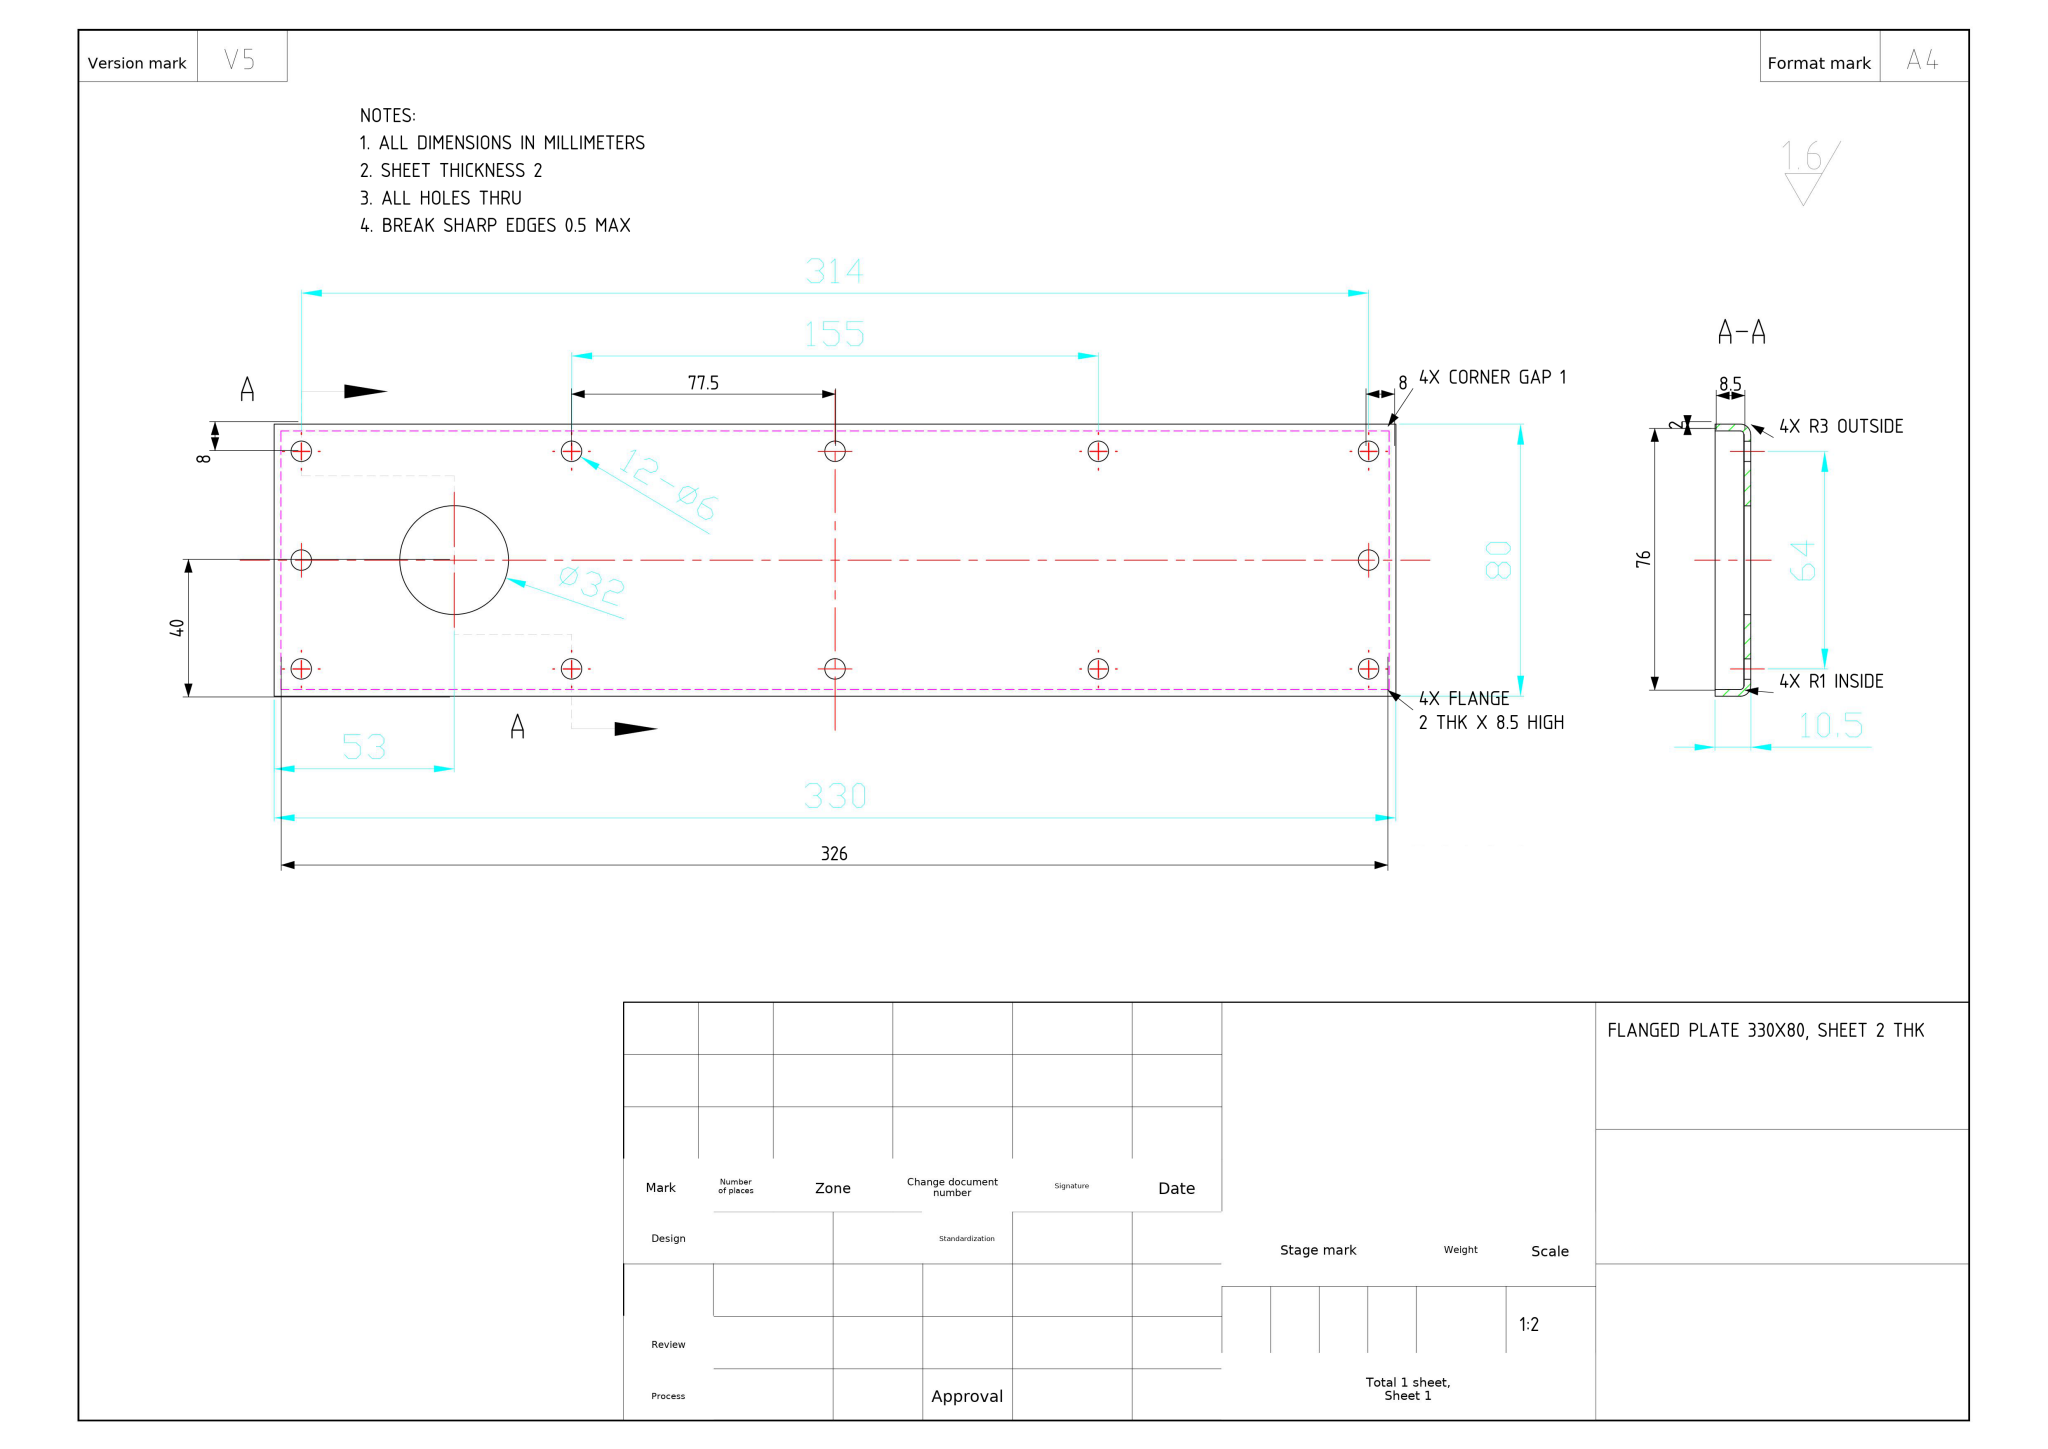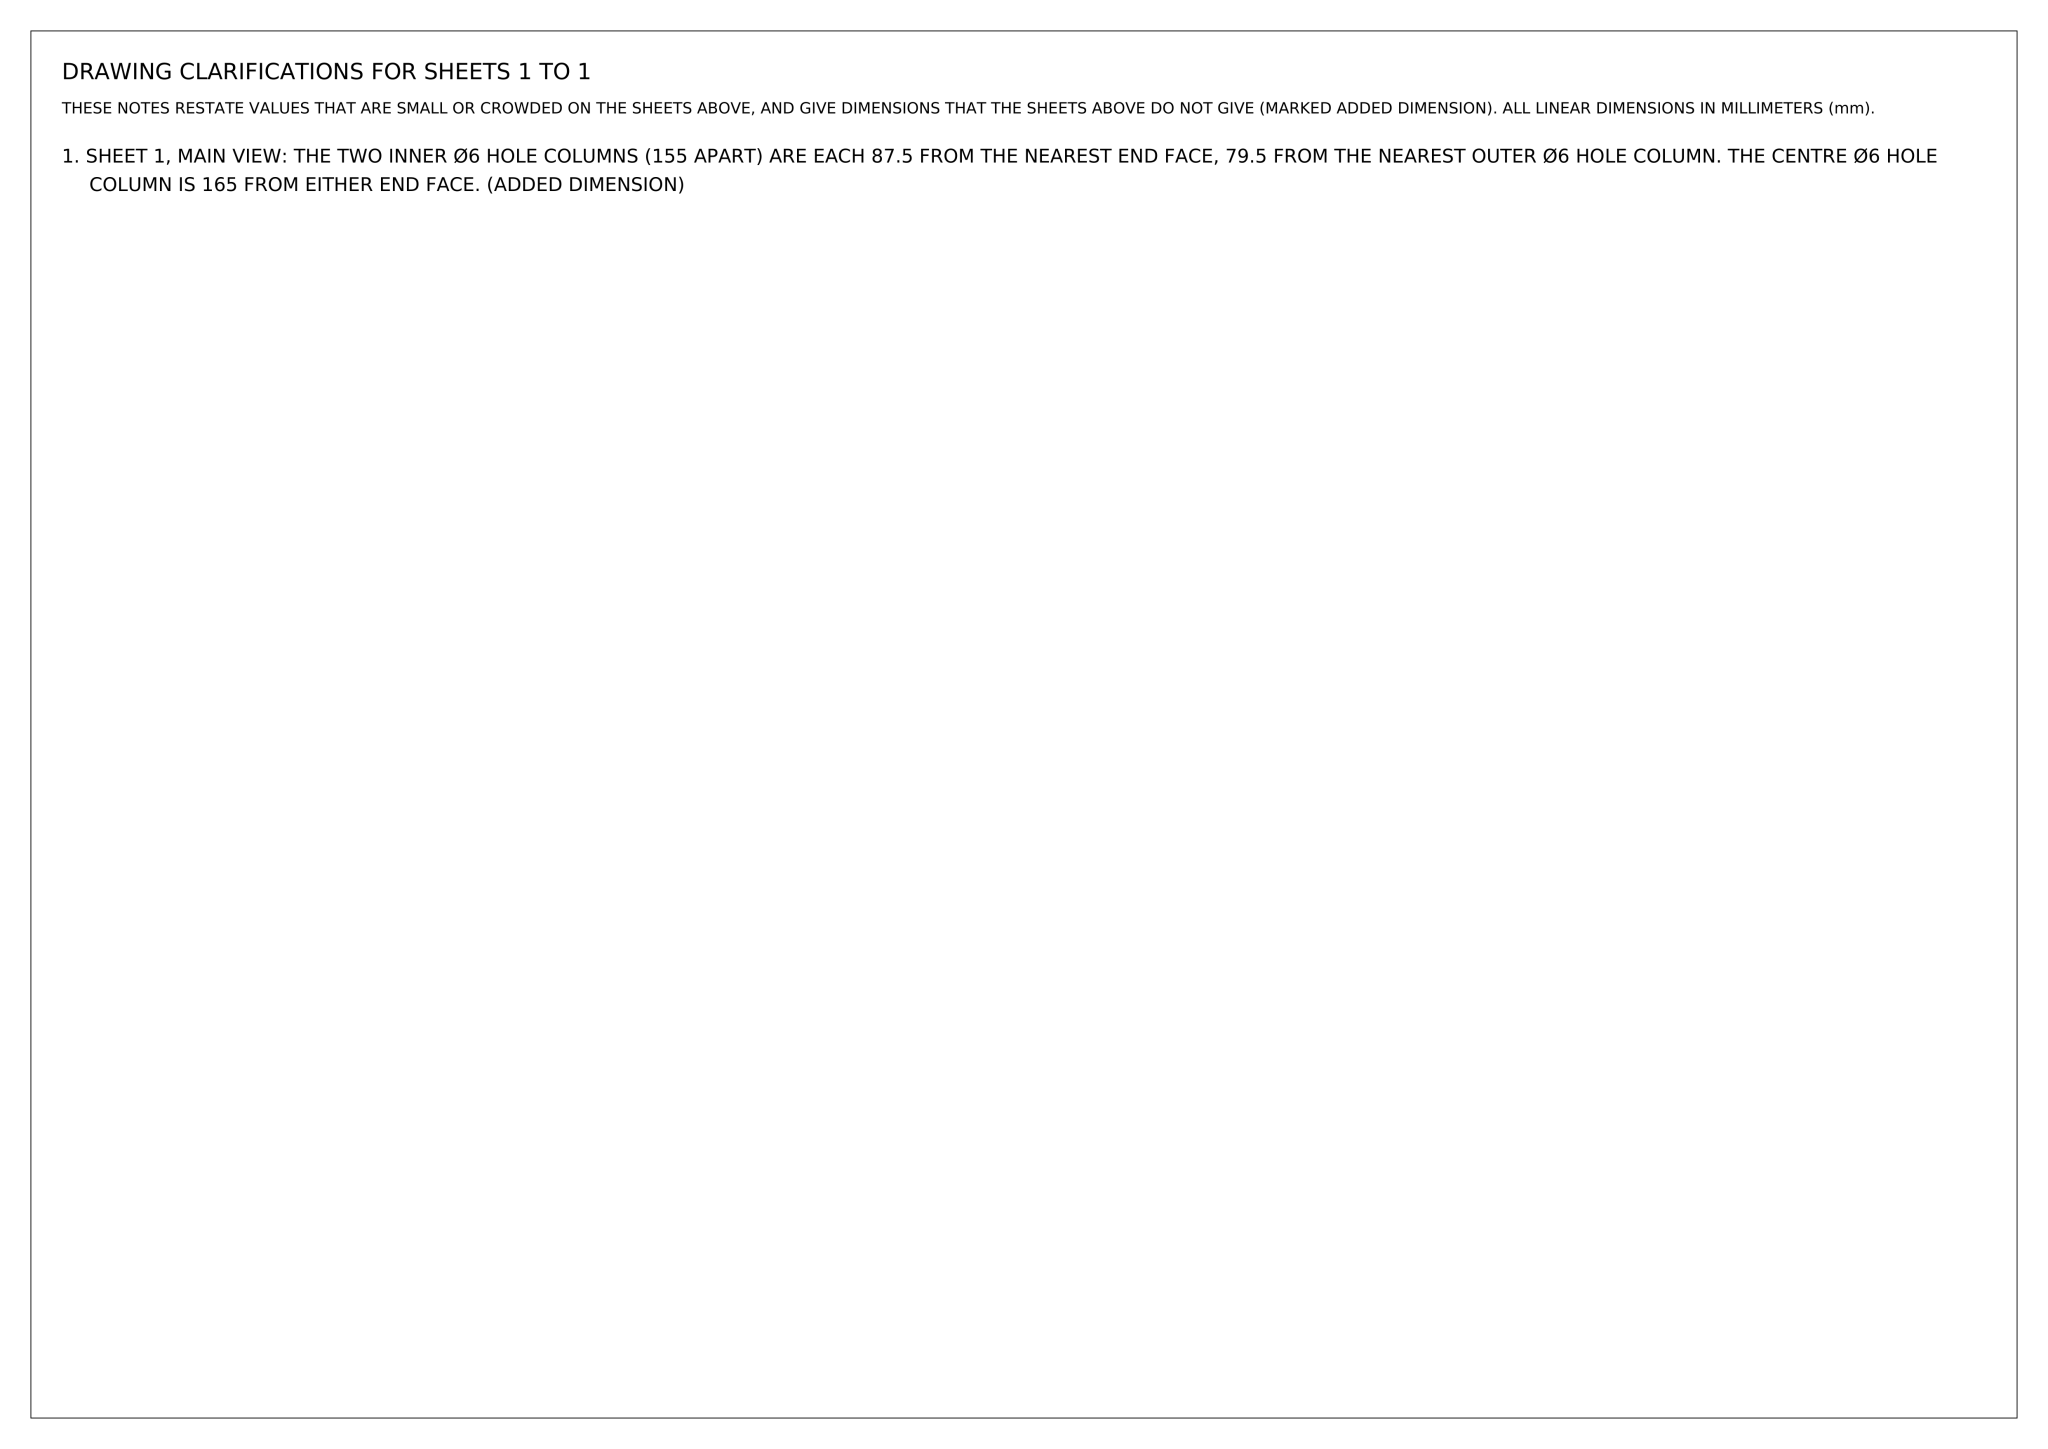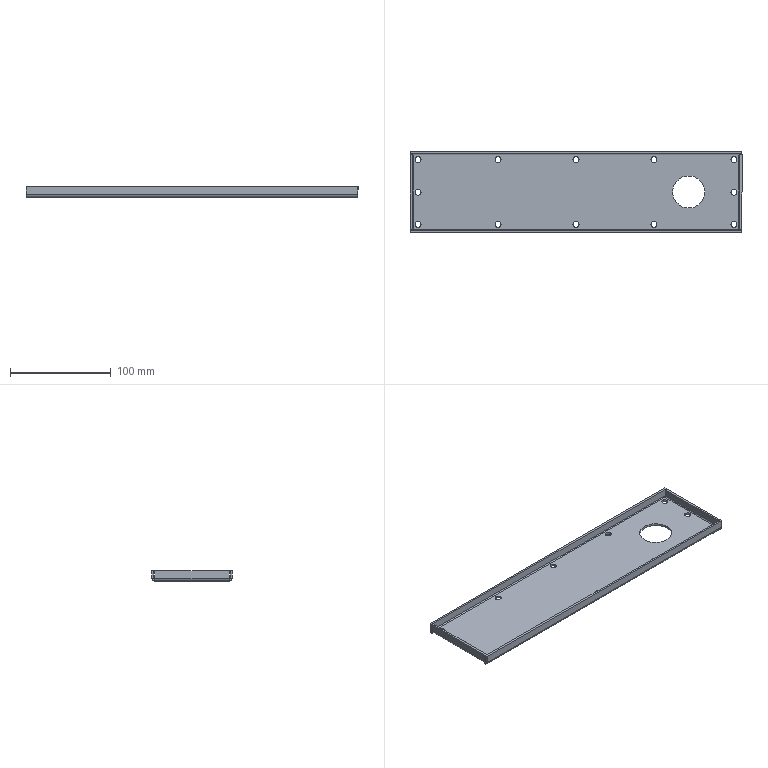Part | NX | mm | 1 solid | 68 faces | box 330 x 80 x 10.5 mm | volume 62862 mm3 | cylinder 34 | plane 34 | commonest cylinder face diameters 6 x28 2 x4 32 x2